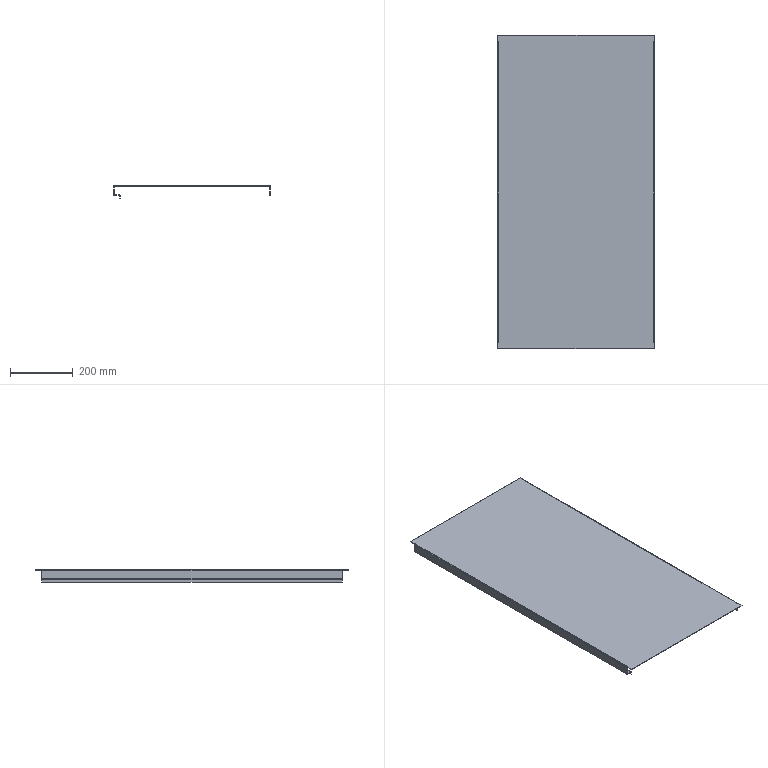Component | SolidWorks | TopPlate-2 | 1 solid | 54 faces | volume 867108 mm3 | plane 46 | cylinder 8 | commonest cylinder face diameters 4.473 x3 1.473 x3 5 x1 2 x1